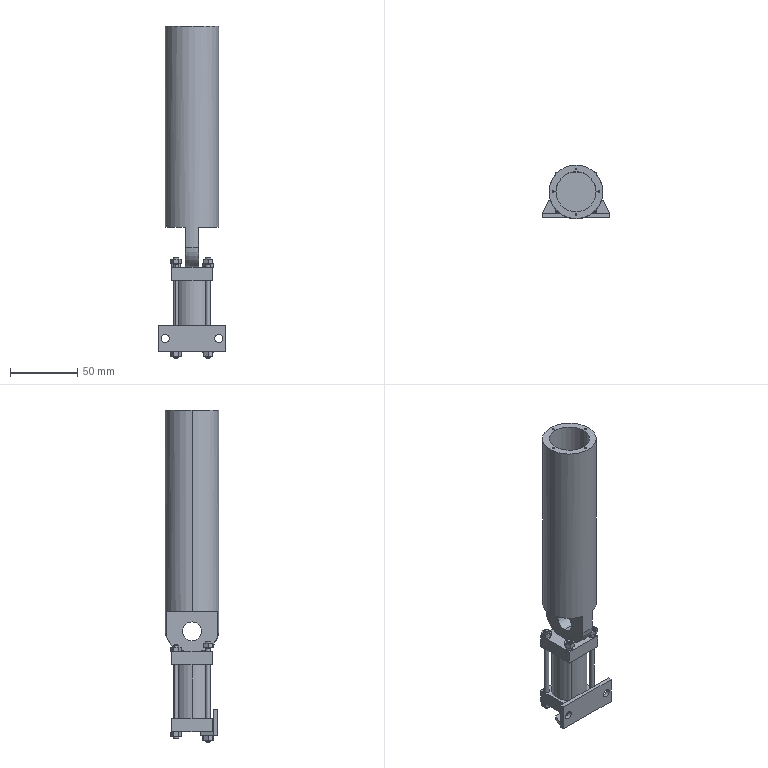Assembly | SolidWorks | mm | 20 component files | 20 solids | 396 faces | box 50 x 40 x 247.54 mm | volume 135687 mm3 | cone 168 | plane 110 | cylinder 100 | torus 18 | commonest cylinder face diameters 4 x32 5 x20 20 x10 1.25 x8 3.464 x8 8 x6 6 x4 21.6 x4
Bill of materials:
Axis | 1 |  | Plain solid cylindrical rod/pin with flat ends; length several times its diameter.
CylinderBody | 1 |  | Hollow cylindrical tube. One end has a flat tang with a rounded end and a single cross-hole; the other end face has four small holes equally spaced.
CylinderFrontCover | 1 |  | Square block with four corner through-holes and a larger central hole. A cylindrical boss on one face has a circumferential groove with a half-round profile.
GB3452.1-92O-ring18x1.8 | 2 |  | Thin torus ring with a round cross-section (O-ring-like shape).
GB_T6170-2000Type1HexNutGradeAAndBM4 | 8 |  | Hexagonal nut-like body with a central round through-bore. The outer corners are chamfered on both faces, and the bore entry is chamfered or countersunk.
GB_T901-1988EqualLengthDoubleEndStudGradeBM4x70 | 2 |  | Long slender cylindrical rod. Short end sections are set off by circumferential step or groove lines, and the ends are chamfered.
GB_T901-1988EqualLengthDoubleEndStudGradeBM4x75 | 2 |  | Long slender cylindrical rod. Short end sections are set off by circumferential step or groove lines, and the ends are chamfered.
CylinderRearCover3 | 1 |  | Square block with four corner through-holes. A raised cylindrical boss on the top face has a central hole and a circumferential groove with a half-round profile.
RoundBarrel | 1 |  | Thick-walled cylindrical sleeve/tube with a plain outer surface and a small internal step or counterbore near one end.
Stand | 1 |  | L-shaped angle bracket. A rectangular upright flange has two round holes. The shorter perpendicular flange has two holes and angled (tapered) side edges.
Mates:
1. concentric | RearEndCapAssembly-1/CylinderRearCover3-1 face at (-5.875, 10.354, -7.5) dir (0, 0, 1) r 2.5 | FrontEndCapAssembly-1/CylinderFrontCover-1 face at (-5.875, 10.354, 37.5) dir (0, 0, 1) r 2.5
2. concentric | FrontEndCapAssembly-1/CylinderFrontCover-1 face at (-5.875, 10.354, 37.5) dir (0, 0, 1) r 2.5 | GB_T901-1988EqualLengthDoubleEndStudGradeBM4x70-1 face at (-5.875, 10.354, -12.516) dir (0, 0, -1) r 1.732
3. concentric | GB_T901-1988EqualLengthDoubleEndStudGradeBM4x70-1 face at (-5.875, 10.354, -12.516) dir (0, 0, -1) r 1.732 | GB_T6170-2000Type1HexNutGradeAAndBM4-1 face at (-5.875, 10.354, -7.5) dir (0, 0, -1) r 2
4. coincident | RearEndCapAssembly-1/CylinderRearCover3-1 face at (-8.875, -16.646, -7.5) dir (0, 0, -1) | GB_T6170-2000Type1HexNutGradeAAndBM4-1 face at (0.7586, 10.327, -7.5) dir (0, 0, 1)
5. concentric | GB_T901-1988EqualLengthDoubleEndStudGradeBM4x70-1 face at (-5.875, 10.354, 57.484) dir (0, 0, 1) r 2 | GB_T6170-2000Type1HexNutGradeAAndBM4-4 face at (-5.875, 10.354, 55.7) dir (0, 0, -1) r 2
6. coincident | FrontEndCapAssembly-1/CylinderFrontCover-1 face at (21.125, -16.646, 52.5) dir (0, 0, 1) | GB_T6170-2000Type1HexNutGradeAAndBM4-4 face at (0.7586, 10.327, 52.5) dir (0, 0, -1)
7. coincident | RearEndCapAssembly-1/CylinderRearCover3-1 face at (-8.875, -16.646, -7.5) dir (0, 0, -1) | Stand-2 face at (-18.875, -17.646, -7.5) dir (0, 0, 1)
8. concentric | RearEndCapAssembly-1/CylinderRearCover3-1 face at (18.125, -13.646, -7.5) dir (0, 0, 1) r 2.5 | Stand-2 face at (18.125, -13.646, -7.5) dir (0, 0, -1) r 2.5
9. concentric | RearEndCapAssembly-1/CylinderRearCover3-1 face at (-5.875, -13.646, -7.5) dir (0, 0, 1) r 2.5 | Stand-2 face at (-5.875, -13.646, -7.5) dir (0, 0, -1) r 2.5
10. concentric | GB_T901-1988EqualLengthDoubleEndStudGradeBM4x75-1 face at (18.125, -13.646, 59.963) dir (0, 0, 1) r 2 | GB_T6170-2000Type1HexNutGradeAAndBM4-6 face at (18.125, -13.646, 58.7) dir (0, 0, -1) r 2
11. coincident | Stand-2 face at (31.125, -17.646, -10.5) dir (0, 0, -1) | GB_T6170-2000Type1HexNutGradeAAndBM4-9 face at (24.759, -13.673, -10.5) dir (0, 0, 1)
12. concentric | GB_T901-1988EqualLengthDoubleEndStudGradeBM4x75-1 face at (18.125, -13.646, -15.037) dir (0, 0, -1) r 2 | GB_T6170-2000Type1HexNutGradeAAndBM4-9 face at (18.125, -13.646, -10.5) dir (0, 0, -1) r 2
13. concentric | FrontEndCapAssembly-1/CylinderFrontCover-1 face at (6.125, -1.646, 52.5) dir (0, 0, -1) r 4 | CylinderBody-1 face at (6.125, -1.646, 232.5) dir (0, 0, -1) r 20
14. coincident | FrontEndCapAssembly-1/CylinderFrontCover-1 face at (21.125, -16.646, 52.5) dir (0, 0, 1) | CylinderBody-1 face at (6.125, -1.646, 52.5) dir (0, 0, -1)
15. concentric | FrontEndCapAssembly-1/CylinderFrontCover-1 face at (6.125, -1.646, 52.5) dir (0, 0, -1) r 4 | RoundBarrel-1 face at (6.125, -1.646, 42.5) dir (0, 0, -1) r 13
16. coincident | RearEndCapAssembly-1/CylinderRearCover3-1 face at (-8.875, -16.646, 2.5) dir (0, 0, 1) | RoundBarrel-1 face at (6.125, -1.646, 2.5) dir (0, 0, -1)
17. concentric | RearEndCapAssembly-1/CylinderRearCover3-1 face at (6.125, -1.646, -2.5) dir (0, 0, 1) r 4 | Axis-1 face at (6.125, -1.646, -2.5) dir (0, 0, 1) r 4
18. coincident | RearEndCapAssembly-1/CylinderRearCover3-1 face at (6.125, -1.646, -2.5) dir (0, 0, 1) | Axis-1 face at (6.125, -1.646, -2.5) dir (0, 0, -1)
19. concentric | CylinderFrontCover-1 face at (2.503, 0.461, -7.5) dir (0, 0, 1) r 4 | GB3452.1-92O-ring18x1.8-1 sketch segment at (2.503, 0.461, 5.1) dir (0, 0, -1) r 9.9
20. coincident | CylinderFrontCover-1 plane at (6.345, 1.722, 6) dir (0, 0, 1) | GB3452.1-92O-ring18x1.8-1 plane at (2.503, 0.461, 6) dir (0, 0, -1)
21. concentric | CylinderRearCover3-1 face at (-0.9879, -0.8562, -2.5) dir (0, 0, 1) r 4 | GB3452.1-92O-ring18x1.8-1 sketch segment at (-0.9879, -0.8562, 5.1) dir (0, 0, -1) r 9.9
22. coincident | CylinderRearCover3-1 plane at (18.164, 0.4047, 6) dir (0, 0, 1) | GB3452.1-92O-ring18x1.8-1 plane at (-0.9879, -0.8562, 6) dir (0, 0, -1)